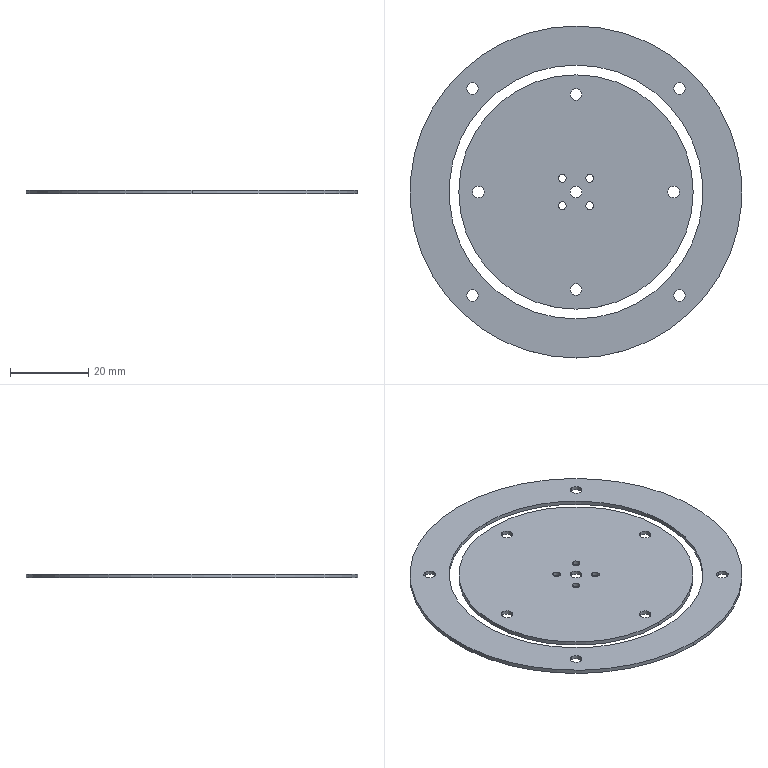Component | SolidWorks | Gimbal-1_Gimbal1-1 | 2 solids | 36 faces | box 85 x 85 x 1 mm | volume 5107 mm3 | cylinder 32 | plane 4 | commonest cylinder face diameters 3 x18 2 x8 65 x2 85 x2 60 x2
build123d program:
from build123d import *

# Parameters (mm, degrees)
SKETCH1_R           = 42.5
BOSS_EXTRUDE1_DEPTH = 1
SKETCH2_R           = 1.5
SKETCH2_R_2         = 1
CUT_EXTRUDE1_DEPTH  = 1
SKETCH3_R           = 32.5
SKETCH3_R_2         = 30
CUT_EXTRUDE2_DEPTH  = 10
SKETCH4_R           = 1.5
CUT_EXTRUDE3_DEPTH  = 10


with BuildPart() as part:
    # Sketch1 → Boss-Extrude1 (new body)
    with BuildSketch(Plane.XY):
        Circle(SKETCH1_R)
    extrude(amount=BOSS_EXTRUDE1_DEPTH)

    # Sketch2 → Cut-Extrude1 (cut)
    with BuildSketch(Plane.XY.offset(1)):
        with Locations((-26.5, 26.5)):
            Circle(SKETCH2_R)
        with Locations(Location((26.5, 26.5, 0), (0, 0, 180))):
            Circle(SKETCH2_R)
        with Locations((26.5, -26.5)):
            Circle(SKETCH2_R)
        with Locations(Location((-26.5, -26.5, 0), (0, 0, 180))):
            Circle(SKETCH2_R)
        Circle(SKETCH2_R)
        with Locations((-3.5, 3.5)):
            Circle(SKETCH2_R_2)
        with Locations((3.5, 3.5)):
            Circle(SKETCH2_R_2)
        with Locations((3.5, -3.5)):
            Circle(SKETCH2_R_2)
        with Locations((-3.5, -3.5)):
            Circle(SKETCH2_R_2)
    extrude(amount=-CUT_EXTRUDE1_DEPTH, mode=Mode.SUBTRACT)

    # Sketch3 → Cut-Extrude2 (cut)
    with BuildSketch(Plane.XY.offset(1)):
        Circle(SKETCH3_R)
        Circle(SKETCH3_R_2, mode=Mode.SUBTRACT)
    extrude(amount=-CUT_EXTRUDE2_DEPTH, mode=Mode.SUBTRACT)


with BuildPart() as cut_extrude2_piece_1:
    # of the separate pieces the step leaves, piece 1, a body of its own (cut_extrude2_pieces)
    add(part.part.solids().sort_by_distance((30, 0, 0))[0])

    # Sketch4 → Cut-Extrude3 (cut)
    with BuildSketch(Plane.XY.offset(1)):
        with Locations((0, 25)):
            Circle(SKETCH4_R)
        with Locations((25, 0)):
            Circle(SKETCH4_R)
        with Locations((0, -25)):
            Circle(SKETCH4_R)
        with Locations((-25, 0)):
            Circle(SKETCH4_R)
    extrude(amount=-CUT_EXTRUDE3_DEPTH, mode=Mode.SUBTRACT)


with BuildPart() as cut_extrude2_piece_2:
    # of the separate pieces the step leaves, piece 2, a body of its own (cut_extrude2_pieces)
    add(part.part.solids().sort_by_distance((42.5, 0, 0))[0])


solid = Compound([cut_extrude2_piece_1.part, cut_extrude2_piece_2.part])

# Placed as in the assembly
solid = solid.moved(Location((0, 96.5, -38), (0, 0, 0)))